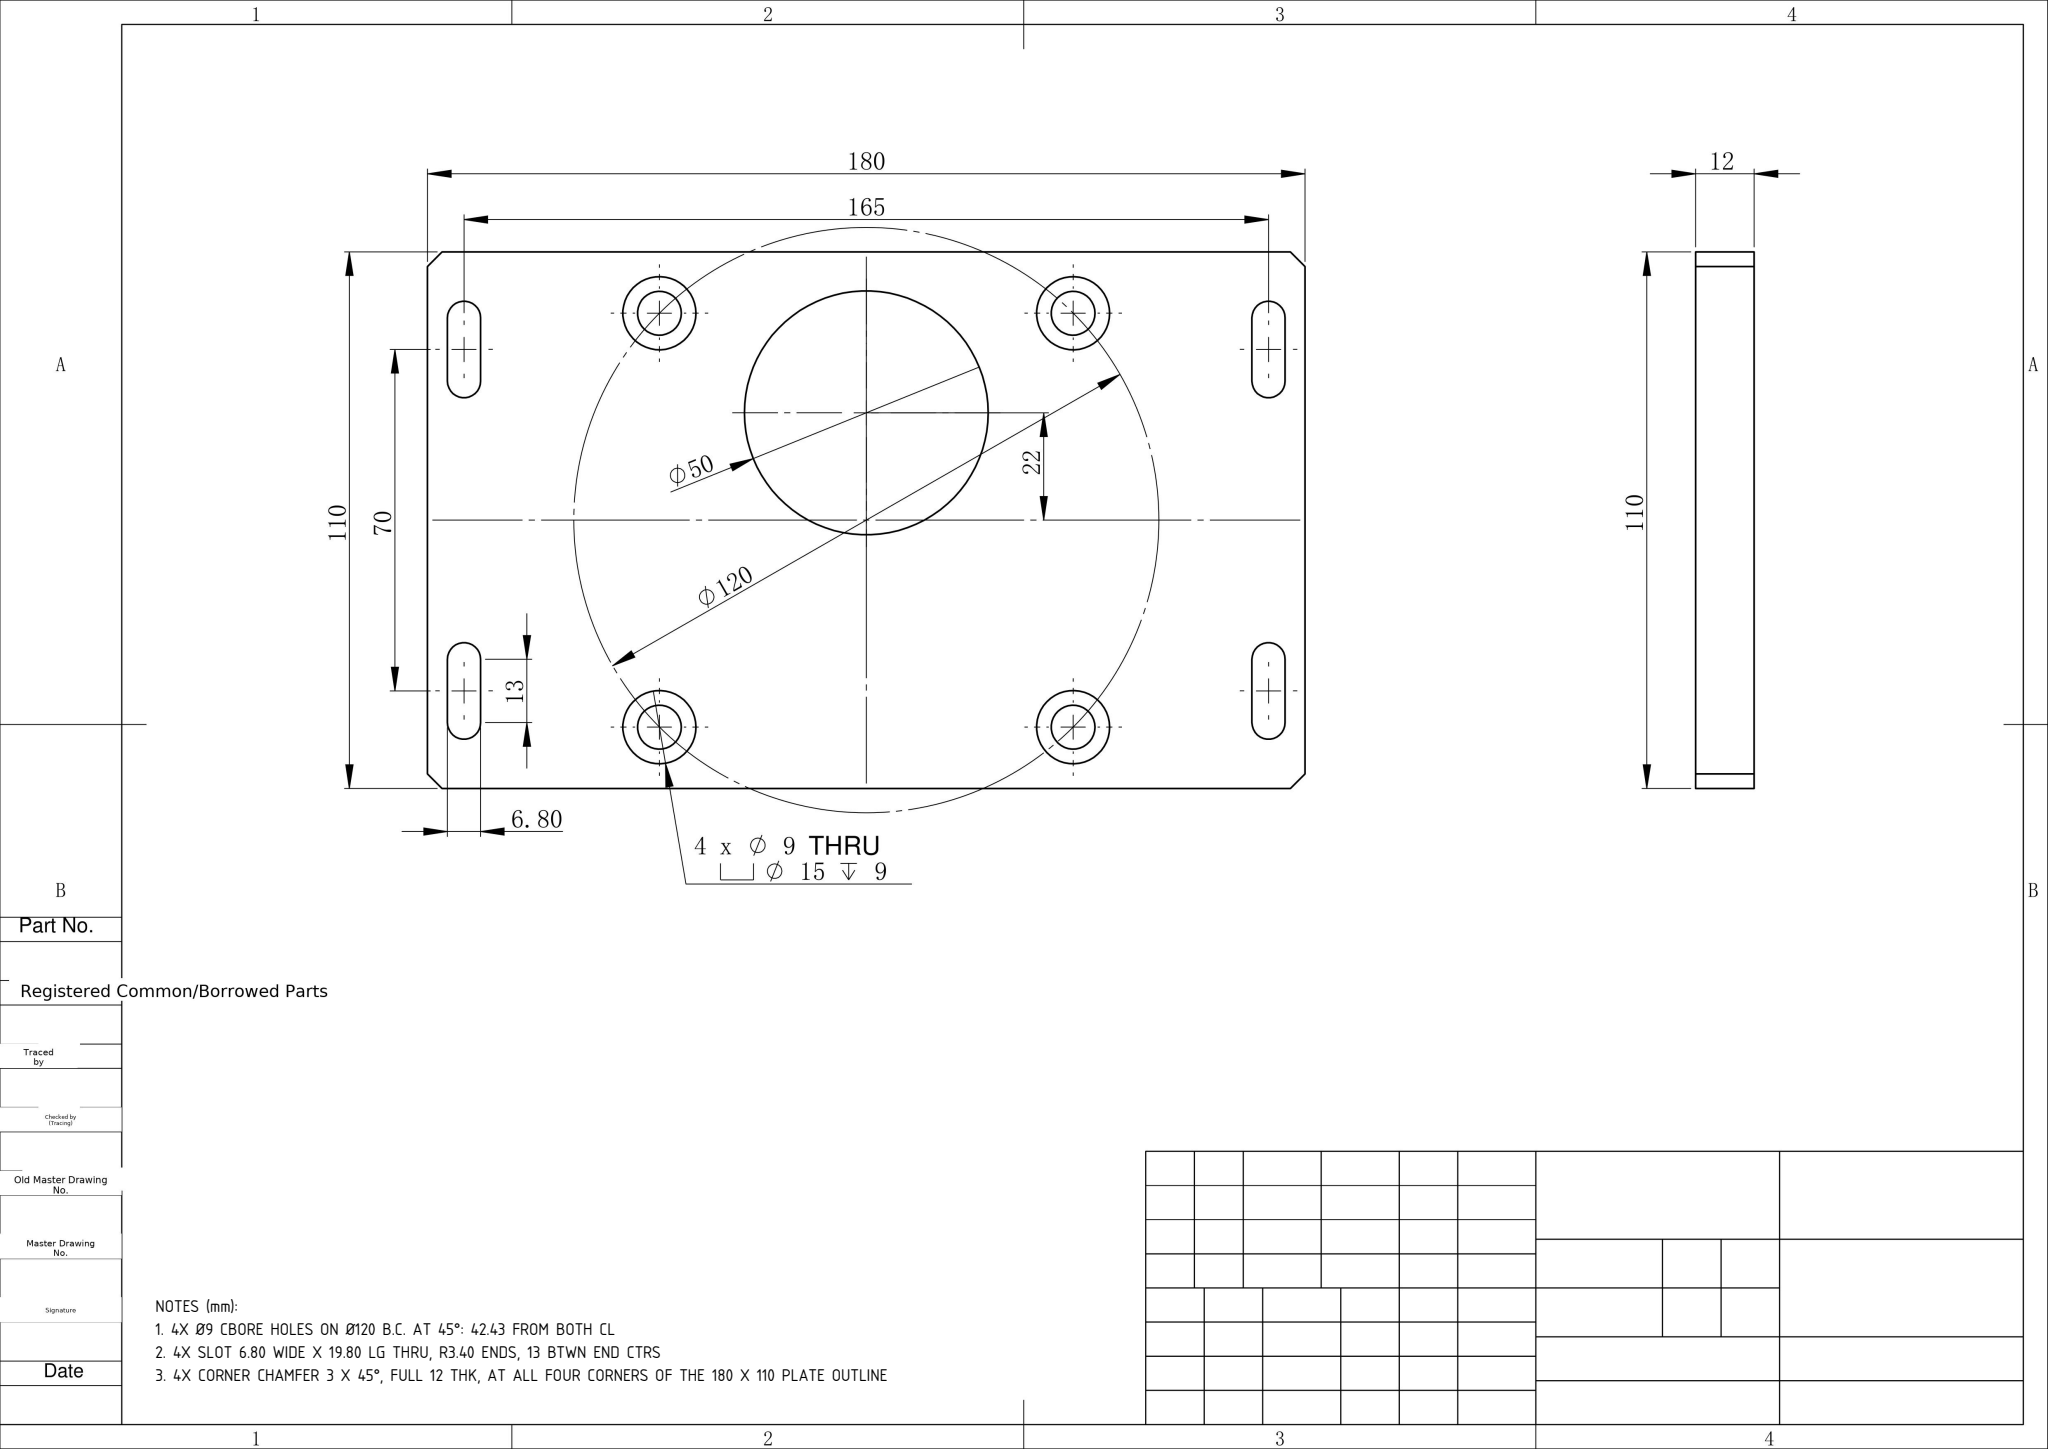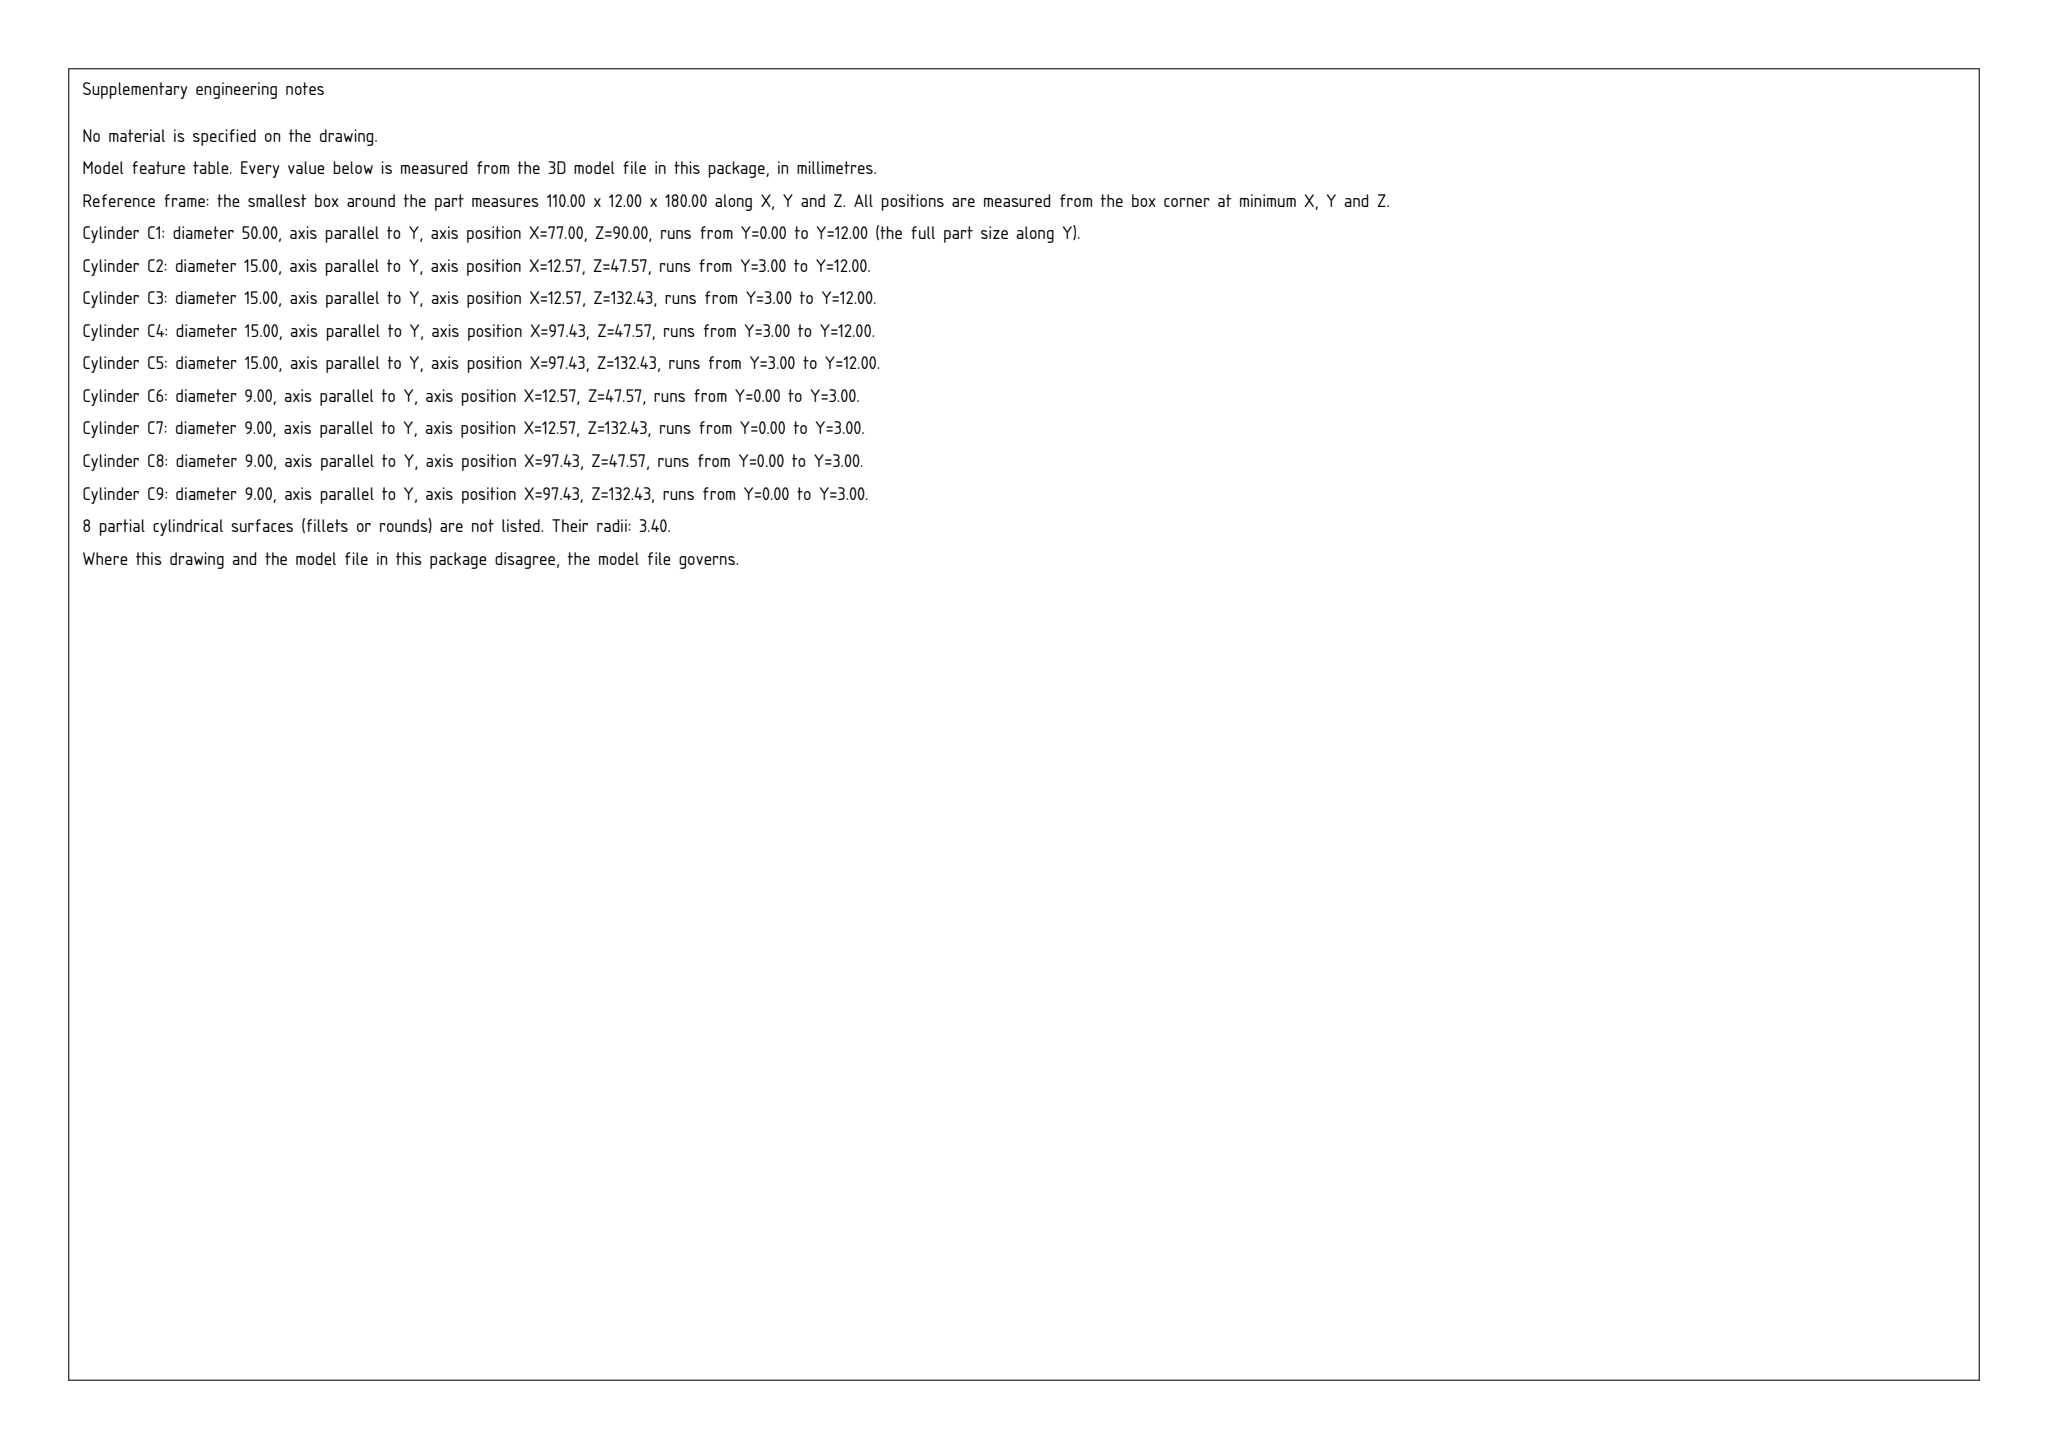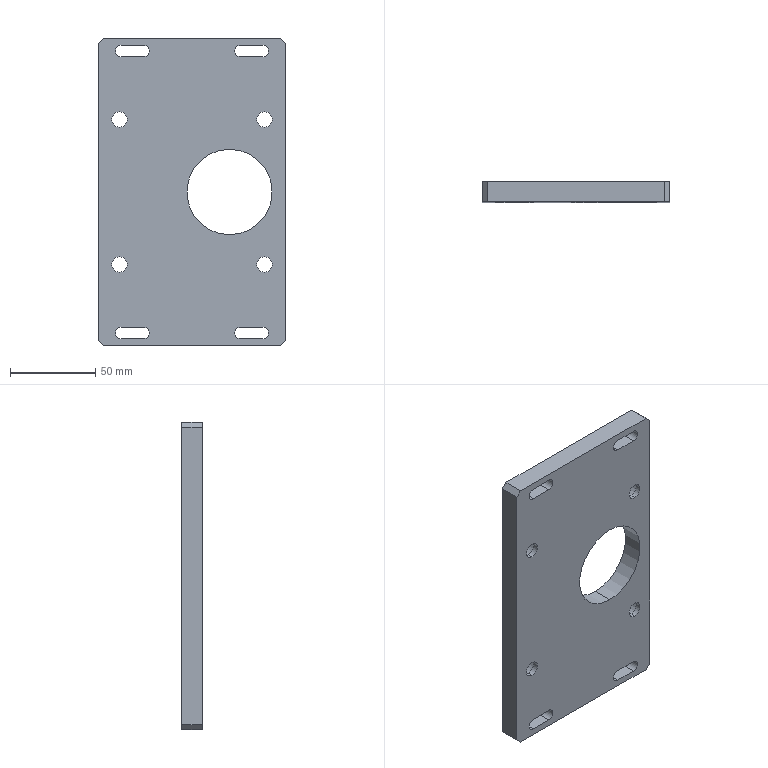Part | SolidWorks | mm | 1 solid | 48 faces | box 110 x 12 x 180 mm | volume 200711 mm3 | cylinder 26 | plane 22 | commonest cylinder face diameters 15 x8 9 x8 6.8 x8 50 x2
Drawing notes:
4X Ø9 CBORE HOLES ON Ø120 B.C. AT 45°: 42.43 FROM BOTH CL | from the solid: Ø9/Ø15 holes at (12.57,47.57),(12.57,132.43),(97.43,47.57),(97.43,132.43); CL (55,90) -> ±42.43, R60 BC
4X SLOT 6.80 WIDE X 19.80 LG THRU, R3.40 ENDS, 13 BTWN END CTRS | from the solid: Ø6.8 thru pairs x=13.5/26.5 & 83.5/96.5 (13 apart) at z=7.5 & 172.5; lg=13+6.8=19.8, R3.4
4X CORNER CHAMFER 3 X 45°, FULL 12 THK, AT ALL FOUR CORNERS OF THE 180 X 110 PLATE OUTLINE | from the solid: inclined_planes(chamfers/angled faces): 4 planes at angle_to_xyz_axes [45,90,45], size [3.0,12.0,3.0], at bbox_from [0,0,0], [0,0,177], [107,0,0], [107,0,177]